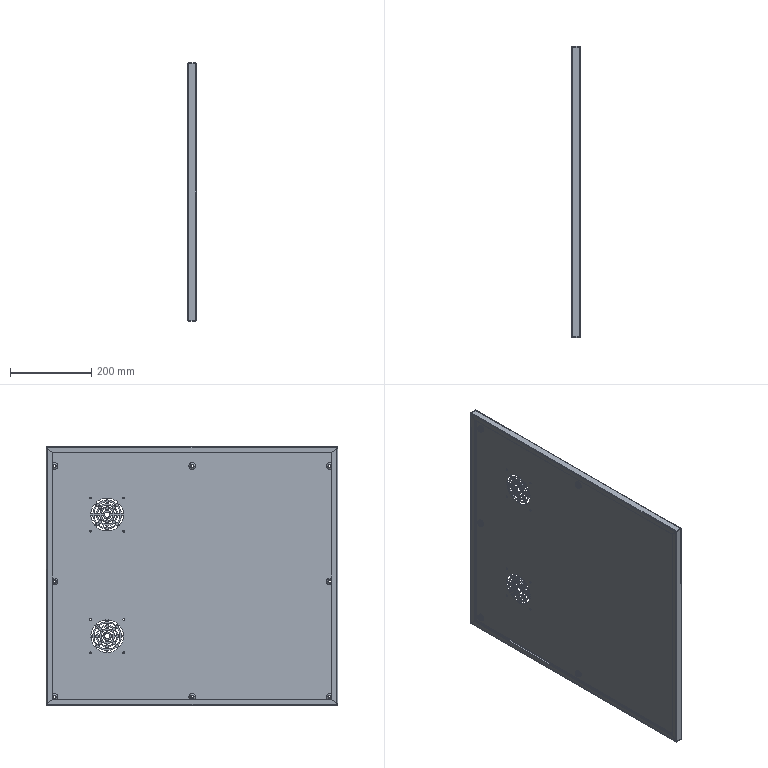Component | SolidWorks | 01-06LeftGuardPlate-1 | 1 solid | 542 faces | volume 800441 mm3 | cylinder 368 | plane 70 | torus 64 | spline 40 | commonest cylinder face diameters 5 x168 4.5 x16 15 x16 12 x16 6.5 x16 71 x16 81 x16 54 x16 | material SPCC